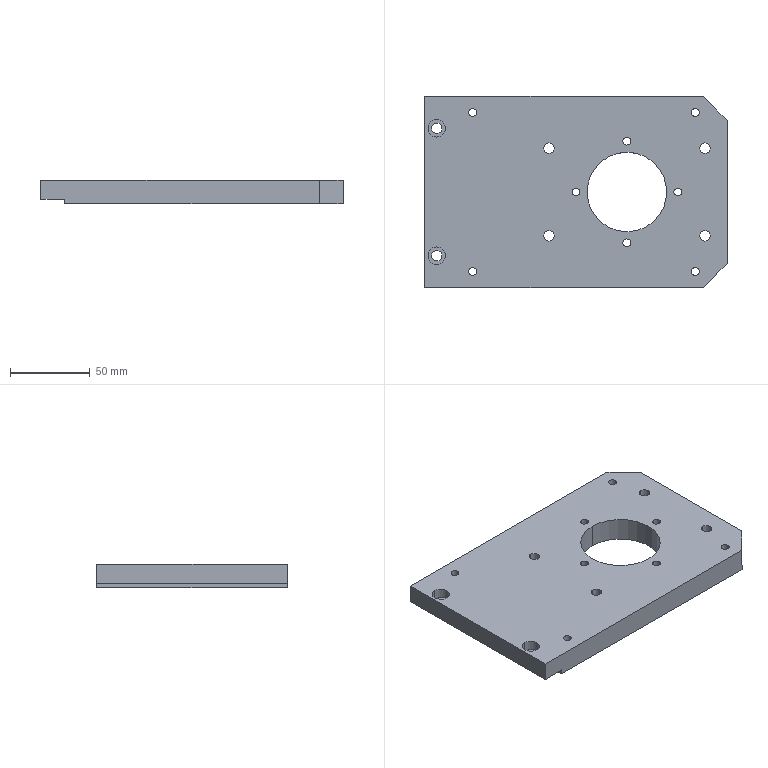Component | SolidWorks | WT-FLD-EJG-1212-00-006-1 | 1 solid | 58 faces | box 190 x 120 x 15 mm | volume 296207 mm3 | cylinder 42 | plane 16 | commonest cylinder face diameters 5 x16 11 x12 6.6 x12 50 x2 | material AISI 1045 Steel, cold drawn
build123d program:
from build123d import *

# Parameters (mm, degrees)
SKETCH1_W                                       = 120
SKETCH1_H                                       = 190
BOSS_EXTRUDE1_DEPTH                             = 15
CHAMFER1_SIZE                                   = 15
SKETCH2_W                                       = 120
SKETCH2_H                                       = 15
CUT_EXTRUDE1_DEPTH                              = 3
M6_HEX_SOCKET_HEAD_CAP_SCREW_CBORE1_D           = 6.6
M6_HEX_SOCKET_HEAD_CAP_SCREW_CBORE1_CBORE_D     = 11
M6_HEX_SOCKET_HEAD_CAP_SCREW_CBORE1_CBORE_DEPTH = 6.4
SKETCH11_R                                      = 25
CUT_EXTRUDE3_DEPTH                              = 200.812
M6_HEX_SOCKET_HEAD_CAP_SCREW_CBORE2_D           = 6.6
M6_HEX_SOCKET_HEAD_CAP_SCREW_CBORE2_CBORE_D     = 11
M6_HEX_SOCKET_HEAD_CAP_SCREW_CBORE2_CBORE_DEPTH = 6.4
M6_TAPPED_HOLE1_D                               = 5
M6_TAPPED_HOLE2_D                               = 5


with BuildPart() as part:
    # Sketch1 → Boss-Extrude1 (new body)
    with BuildSketch(Plane.XY):
        with Locations((0, 95)):
            Rectangle(SKETCH1_W, SKETCH1_H)
    extrude(amount=BOSS_EXTRUDE1_DEPTH)

    # Chamfer1
    chamfer1_edges = [part.edges().sort_by_distance(p)[0] for p in [
        (-60, 190, 7.5),
        (60, 190, 7.5),
    ]]
    chamfer(chamfer1_edges, length=CHAMFER1_SIZE)

    # Sketch2 → Cut-Extrude1 (cut)
    with BuildSketch(Plane.XY.offset(15)):
        with Locations((0, 7.5)):
            Rectangle(SKETCH2_W, SKETCH2_H)
    extrude(amount=-CUT_EXTRUDE1_DEPTH, mode=Mode.SUBTRACT)

    # M6 Hex Socket Head Cap Screw CBORE1 (through all)
    with Locations(Plane(origin=(0, 0, 0), x_dir=(-1, 0, 0), z_dir=(0, 0, -1))):
        with Locations((40, 7.5), (-40, 7.5)):
            CounterBoreHole(M6_HEX_SOCKET_HEAD_CAP_SCREW_CBORE1_D / 2, M6_HEX_SOCKET_HEAD_CAP_SCREW_CBORE1_CBORE_D / 2, M6_HEX_SOCKET_HEAD_CAP_SCREW_CBORE1_CBORE_DEPTH)

    # Sketch11 → Cut-Extrude3 (cut, through all)
    with BuildSketch(Plane(origin=(0, 0, 0), x_dir=(-1, 0, 0), z_dir=(0, 0, -1))):
        with Locations((0, 127)):
            Circle(SKETCH11_R)
    extrude(amount=-CUT_EXTRUDE3_DEPTH, mode=Mode.SUBTRACT)

    # M6 Hex Socket Head Cap Screw CBORE2 (through all)
    with Locations(Plane.XY.offset(15)):
        with Locations((27.5, 176), (-27.5, 176), (27.5, 78), (-27.5, 78)):
            CounterBoreHole(M6_HEX_SOCKET_HEAD_CAP_SCREW_CBORE2_D / 2, M6_HEX_SOCKET_HEAD_CAP_SCREW_CBORE2_CBORE_D / 2, M6_HEX_SOCKET_HEAD_CAP_SCREW_CBORE2_CBORE_DEPTH)

    # M6 Tapped Hole1 (through all)
    with Locations(Plane(origin=(0, 0, 0), x_dir=(-1, 0, 0), z_dir=(0, 0, -1))):
        with Locations((-32, 127), (0, 95), (32, 127), (0, 159)):
            Hole(M6_TAPPED_HOLE1_D / 2)

    # M6 Tapped Hole2 (through all)
    with Locations(Plane(origin=(0, 0, 0), x_dir=(-1, 0, 0), z_dir=(0, 0, -1))):
        with Locations((-50, 30), (50, 30), (-50, 170), (50, 170)):
            Hole(M6_TAPPED_HOLE2_D / 2)


solid = part.part

# Placed as in the assembly
solid = solid.moved(Location((-127, 0, 60), (180, 0, -90)))